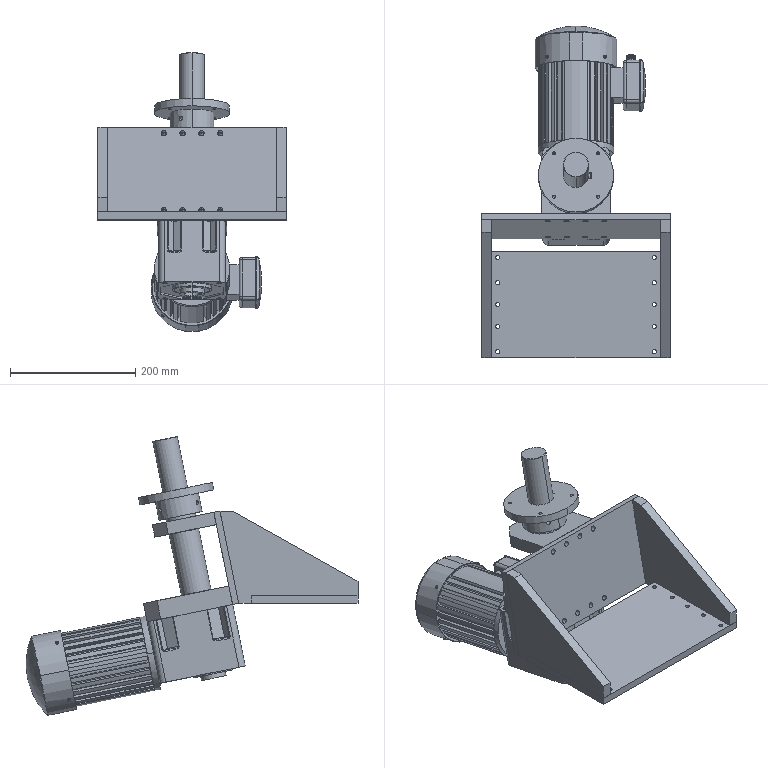Assembly | SolidWorks | mm | 13 component files | 14 solids | 1141 faces | box 300 x 529.19 x 444.46 mm | volume 5927936 mm3 | cylinder 537 | plane 469 | cone 68 | torus 32 | spline 29 | sphere 6 | commonest cylinder face diameters 8.5 x184 5 x56 120 x40 4 x40 6.5 x32 6.8 x22 11 x20 6.6 x20
Bill of materials:
B6008ZZ | 2 |  | Flat annular ring: a short cylinder with a large central through-bore and slightly rounded or chamfered outer edges. Its proportions resemble a ring or rolling-bearing envelope.
HGF2_S400M | 1 |  | Looks like a right-angle gearmotor. A cylindrical body with axial fins and a domed end cap is joined to a boxy housing. The housing has a hollow bore with a keyway that runs perpendicular to the cylinder axis. A small rectangular box sticks out from the side of the cylindrical body.
JL001-04-01-001 | 1 |  | Thin flat rectangular plate with two columns of small round through-holes along each short edge, 20 holes in total. The central field has no features.
JL001-04-01-002 | 1 |  | Thick flat rectangular plate with through-holes: a row of 4 larger holes in the middle area along each long edge, plus 3 smaller holes along each short edge, including the corners.
JL001-04-01-003 | 2 |  | Flat plate with a constant thickness and a roughly triangular, gusset-like outline: a long sloped hypotenuse edge, a short vertical end face at the low end, and a small rectangular step or tab at the bottom of the tall end.
JL001-04-01-004 | 1 |  | Thick block with a single-sided outline: rectangular body with two chamfered corners on one end. It has a large through-bore with an internal step or shoulder (counterbore) and a row of 4 small holes in one side face.
JL001-04-01-005 | 1 |  | Stepped cylindrical shaft with several diameter sections: a long main section, a wider collar or shoulder, a short intermediate step, and a narrower end journal. Small flat or keyway-like recesses sit on two of the sections.
JL001-04-01-006 | 1 |  | Thick block with a single-sided outline: rectangular body with two chamfered corners on one end. It has one large plain circular through-bore and a row of 4 small holes in the side face opposite the chamfered end.
JL001-04-01-007 | 1 |  | Flanged hub: a thin circular flange with 4 small through-holes, joined to a coaxial cylindrical boss and a smaller-diameter stepped end. A central bore with a keyway runs through it, and there is a radial hole in the boss.
Key_10-40 | 1 |  | A solid rectangular bar with both ends fully rounded, giving a stadium-shaped (obround) outline in plan. The edges appear lightly chamfered or rounded. It looks like a round-ended parallel key.
Key_8-50 | 1 |  | A solid rectangular bar with both ends fully rounded, giving a stadium-shaped (obround) outline in plan, with lightly broken edges. It looks like a round-ended parallel key and is more slender than the other bar.
Mates:
1. coincident | JL001-04-01-001-1 face at (-150, 85, 12) dir (0, 1, 0) | JL001-04-01-003-1 face at (135, 85, 0) dir (0, -1, 0)
2. coincident | JL001-04-01-001-1 face at (-150, 85, 12) dir (0, 1, 0) | JL001-04-01-003-2 face at (-150, 85, 0) dir (0, -1, 0)
3. coincident | JL001-04-01-001-1 face at (0, 0, 12) dir (0, 0, 1) | JL001-04-01-003-1 face at (135, 85, 12) dir (0, 0, -1)
4. coincident | JL001-04-01-001-1 face at (0, 0, 12) dir (0, 0, 1) | JL001-04-01-003-2 face at (-150, 85, 12) dir (0, 0, -1)
5. coincident | JL001-04-01-002-1 face at (0, 119.997, 73.485) dir (0, -0.9798, 0.2) | JL001-04-01-003-1 face at (135, 135, 147) dir (0, 0.9798, -0.2)
6. coincident | JL001-04-01-002-1 face at (150, 114.798, -2) dir (1, 0, 0) | JL001-04-01-003-1 face at (150, 135, 0) dir (1, 0, 0)
7. coincident | JL001-04-01-002-1 face at (-150, 114.798, -2) dir (-1, 0, 0) | JL001-04-01-003-2 face at (-150, 135, 0) dir (-1, 0, 0)
8. coincident | JL001-04-01-002-1 edge at (150, 105, 0) dir (-1, 0, 0) | JL001-04-01-003-1 face at (150, 135, 0) dir (0, 0, -1)
9. coincident | JL001-04-01-002-1 face at (0, 129.795, 71.486) dir (0, 0.9798, -0.2) | JL001-04-01-006-1 face at (55, 140.793, 125.375) dir (0, -0.9798, 0.2)
10. coincident | JL001-04-01-002-1 face at (0, 129.795, 71.486) dir (0, 0.9798, -0.2) | JL001-04-01-004-2 face at (-55, 120.797, 27.395) dir (0, -0.9798, 0.2)
11. coincident | JL001-04-01-002-1 face at (-150, 114.798, -2) dir (0, -0.2, -0.9798) | JL001-04-01-004-2 face at (0, 182.894, -15.897) dir (0, -0.2, -0.9798)
12. width | JL001-04-01-004-2 face at (55, 256.99, -0.3999) dir (1, 0, 0) | JL001-04-01-004-2 face at (-55, 256.99, -0.3999) dir (-1, 0, 0) | JL001-04-01-002-1 face at (-150, 114.798, -2) dir (-1, 0, 0) | JL001-04-01-002-1 face at (150, 114.798, -2) dir (1, 0, 0)
13. coincident | JL001-04-01-002-1 face at (-150, 144.792, 144.971) dir (0, 0.2, 0.9798) | JL001-04-01-006-1 face at (0, 193.782, 134.973) dir (0, 0.2, 0.9798)
14. width | JL001-04-01-006-1 face at (55, 238.773, 105.379) dir (1, 0, 0) | JL001-04-01-006-1 face at (-55, 238.773, 105.379) dir (-1, 0, 0) | JL001-04-01-002-1 face at (-150, 114.798, -2) dir (-1, 0, 0) | JL001-04-01-002-1 face at (150, 114.798, -2) dir (1, 0, 0)
15. concentric | JL001-04-01-004-2 face at (0, 169.727, 2.1) dir (0, 0.2, 0.9798) r 34 | B6008ZZ-2 face at (0, 172.726, 16.797) dir (0, -0.2, -0.9798) r 34
16. concentric | JL001-04-01-006-1 face at (0, 195.722, 129.474) dir (0, -0.2, -0.9798) r 34 | B6008ZZ-1 face at (0, 192.722, 114.777) dir (0, 0.2, 0.9798) r 34
17. coincident | JL001-04-01-006-1 face at (0, 195.722, 129.474) dir (0, -0.2, -0.9798) | B6008ZZ-1 face at (5.425, 227.615, 122.965) dir (0, 0.2, 0.9798)
18. coincident | JL001-04-01-004-2 face at (0, 169.727, 2.1) dir (0, 0.2, 0.9798) | B6008ZZ-2 face at (-20.28, 195.234, -3.106) dir (0, -0.2, -0.9798)
19. width | JL001-04-01-002-1 face at (150, 114.798, -2) dir (1, 0, 0) | JL001-04-01-002-1 face at (-150, 114.798, -2) dir (-1, 0, 0) | JL001-04-01-001-1 face at (-150, 85, 12) dir (-1, 0, 0) | JL001-04-01-001-1 face at (150, 85, 12) dir (1, 0, 0)
20. concentric | B6008ZZ-2 face at (0, 172.726, 16.797) dir (0, -0.2, -0.9798) r 20 | JL001-04-01-005-1 face at (0, 222.716, 261.748) dir (0, 0.2, 0.9798) r 20
21. coincident | B6008ZZ-2 face at (-12.906, 188.958, 13.484) dir (0, 0.2, 0.9798) | JL001-04-01-005-1 face at (24, 172.726, 16.797) dir (0, -0.2, -0.9798)
22. concentric | JL001-04-01-005-1 face at (0, 222.716, 261.748) dir (0, 0.2, 0.9798) r 12.5 | HGF2_S400M-1 face at (0, 168.527, -3.779) dir (0, -0.2, -0.9798) r 12.5
23. coincident | JL001-04-01-004-2 face at (0, 182.894, -15.897) dir (0, -0.2, -0.9798) | HGF2_S400M-1 face at (53.5, 250.991, -29.794) dir (0, 0.2, 0.9798)
24. width | HGF2_S400M-1 face at (53.5, 250.991, -29.794) dir (1, 0, 0) | HGF2_S400M-1 face at (-53.5, 250.991, -29.794) dir (-1, 0, 0) | JL001-04-01-004-2 face at (-55, 256.99, -0.3999) dir (-1, 0, 0) | JL001-04-01-004-2 face at (55, 256.99, -0.3999) dir (1, 0, 0)
25. coincident | JL001-04-01-005-1 face at (8.5, 168.727, -2.799) dir (1, 0, 0) | Key_8-50-1 face at (8.5, 165.608, 1.92) dir (-1, 0, 0)
26. concentric | JL001-04-01-005-1 face at (18.5, 168.727, -2.799) dir (-1, 0, 0) r 4 | Key_8-50-1 face at (8.5, 168.727, -2.799) dir (1, 0, 0) r 4
27. coincident | JL001-04-01-005-1 face at (18.5, 164.808, -2) dir (0, 0.9798, -0.2) | Key_8-50-1 face at (8.5, 165.608, 1.92) dir (0, -0.9798, 0.2)
28. coincident | JL001-04-01-005-1 face at (15, 204.72, 173.565) dir (1, 0, 0) | Key_10-40-1 face at (15, 201.621, 133.373) dir (-1, 0, 0)
29. concentric | JL001-04-01-005-1 face at (25, 197.721, 139.272) dir (-1, 0, 0) r 5 | Key_10-40-1 face at (15, 197.721, 139.272) dir (1, 0, 0) r 5
30. coincident | JL001-04-01-005-1 face at (25, 199.821, 174.565) dir (0, 0.9798, -0.2) | Key_10-40-1 face at (15, 191.823, 135.373) dir (0, -0.9798, 0.2)
31. concentric | JL001-04-01-005-1 face at (0, 222.716, 261.748) dir (0, 0.2, 0.9798) r 20 | JL001-04-01-007-1 face at (0, 195.722, 129.474) dir (0, -0.2, -0.9798) r 20
32. coincident | B6008ZZ-1 face at (3.88, 218.531, 124.819) dir (0, 0.2, 0.9798) | JL001-04-01-007-1 face at (20, 195.722, 129.474) dir (0, -0.2, -0.9798)
33. coincident | Key_10-40-1 face at (15, 201.621, 133.373) dir (0, 0.9798, -0.2) | JL001-04-01-007-1 face at (25, 200.621, 128.474) dir (0, -0.9798, 0.2)